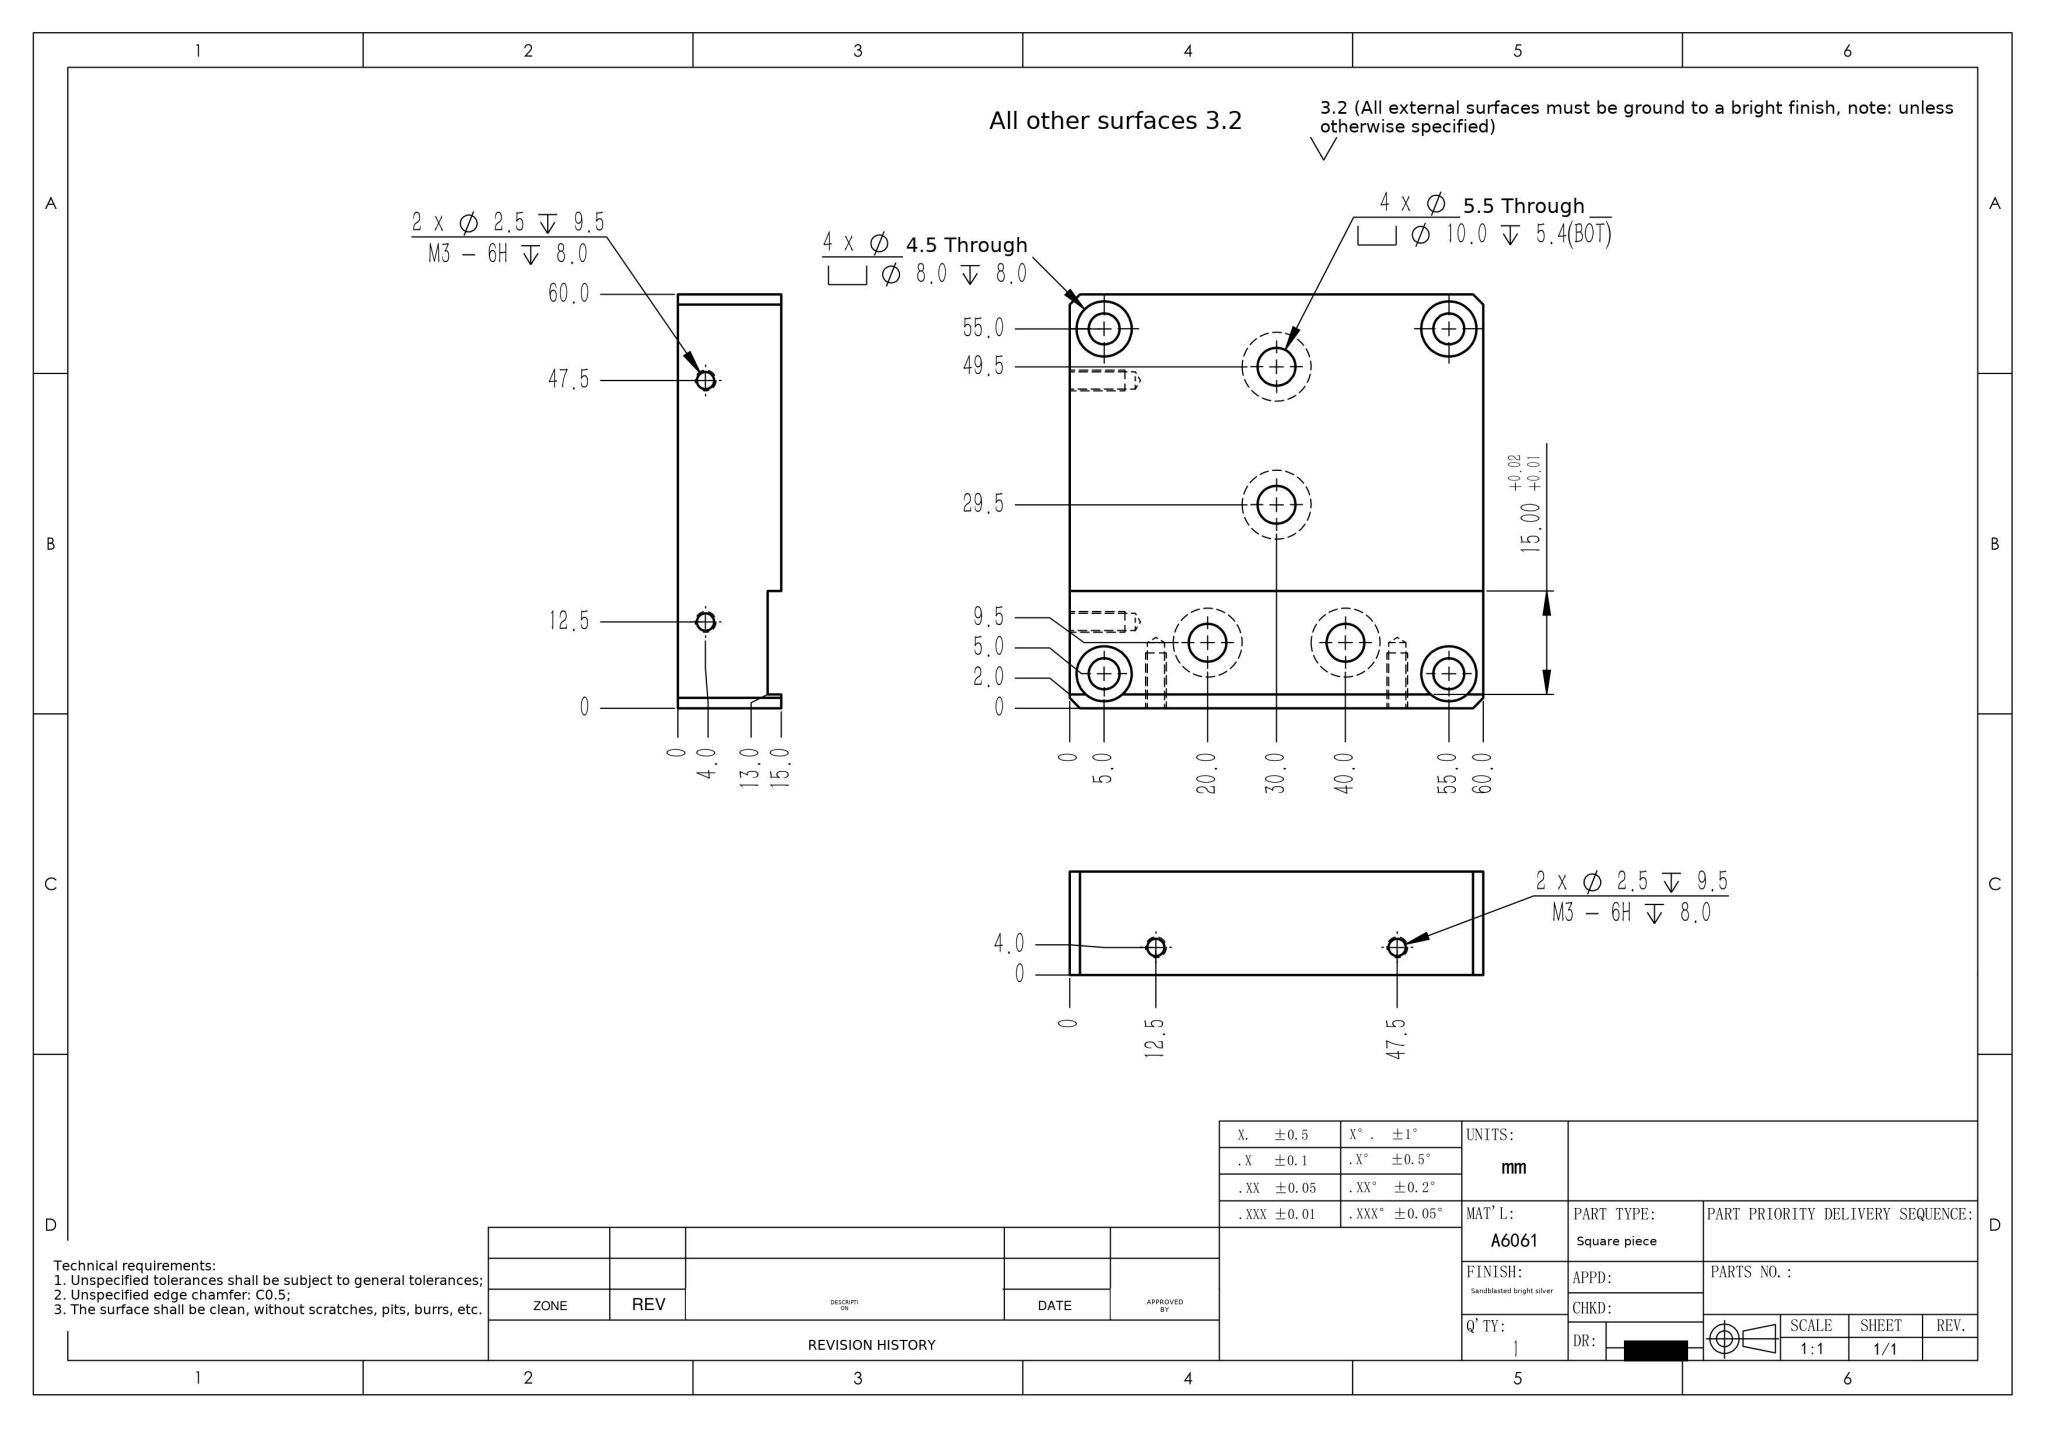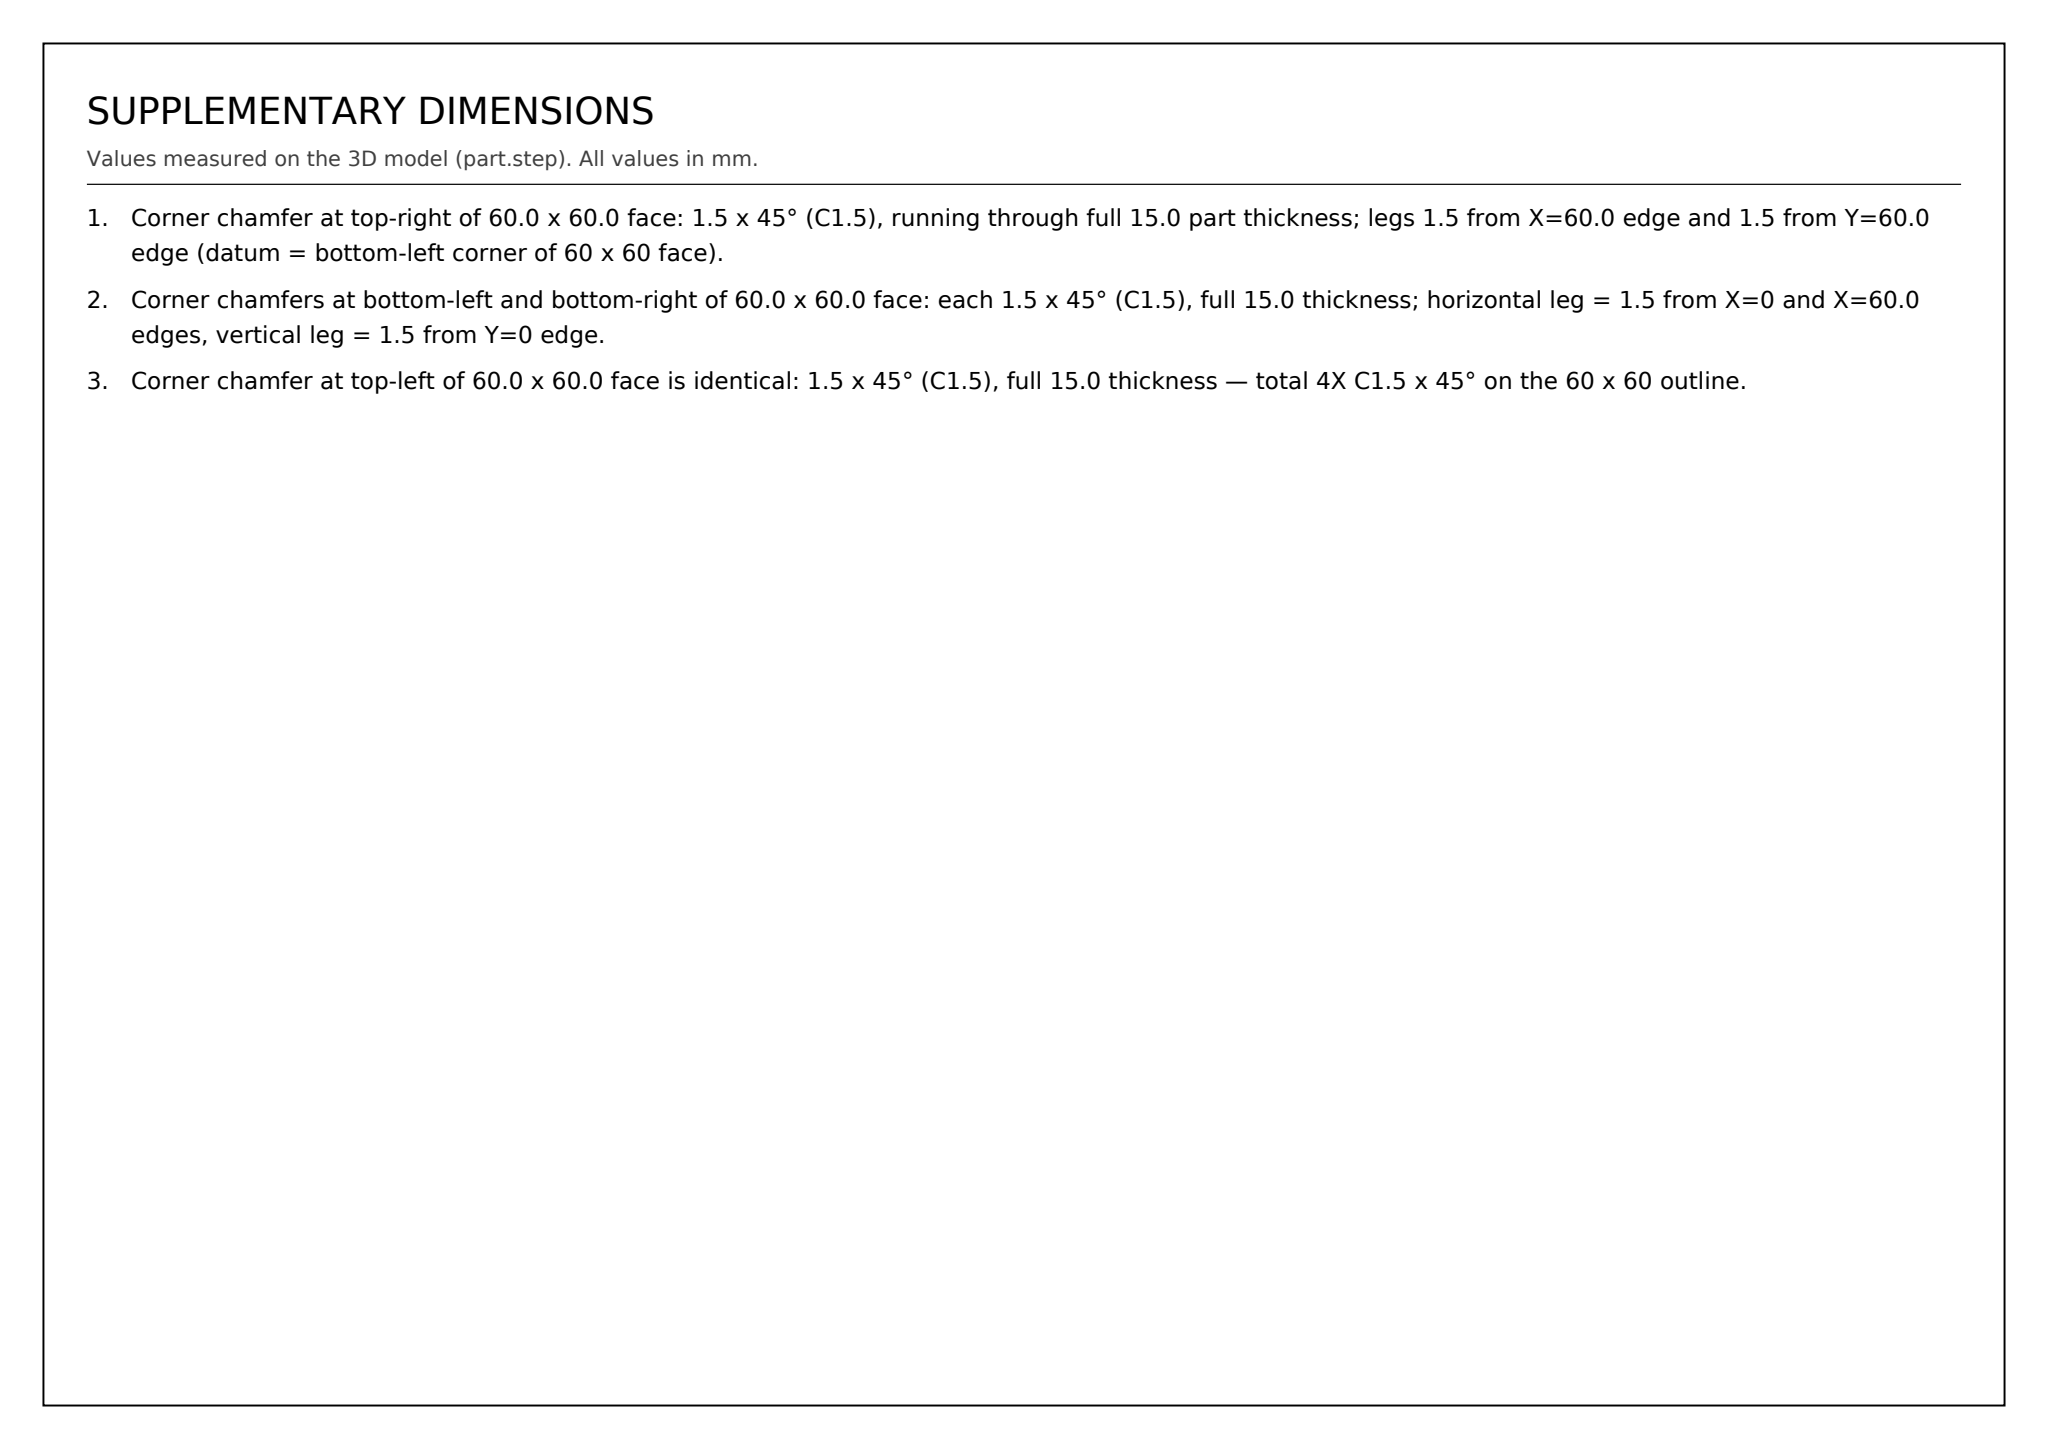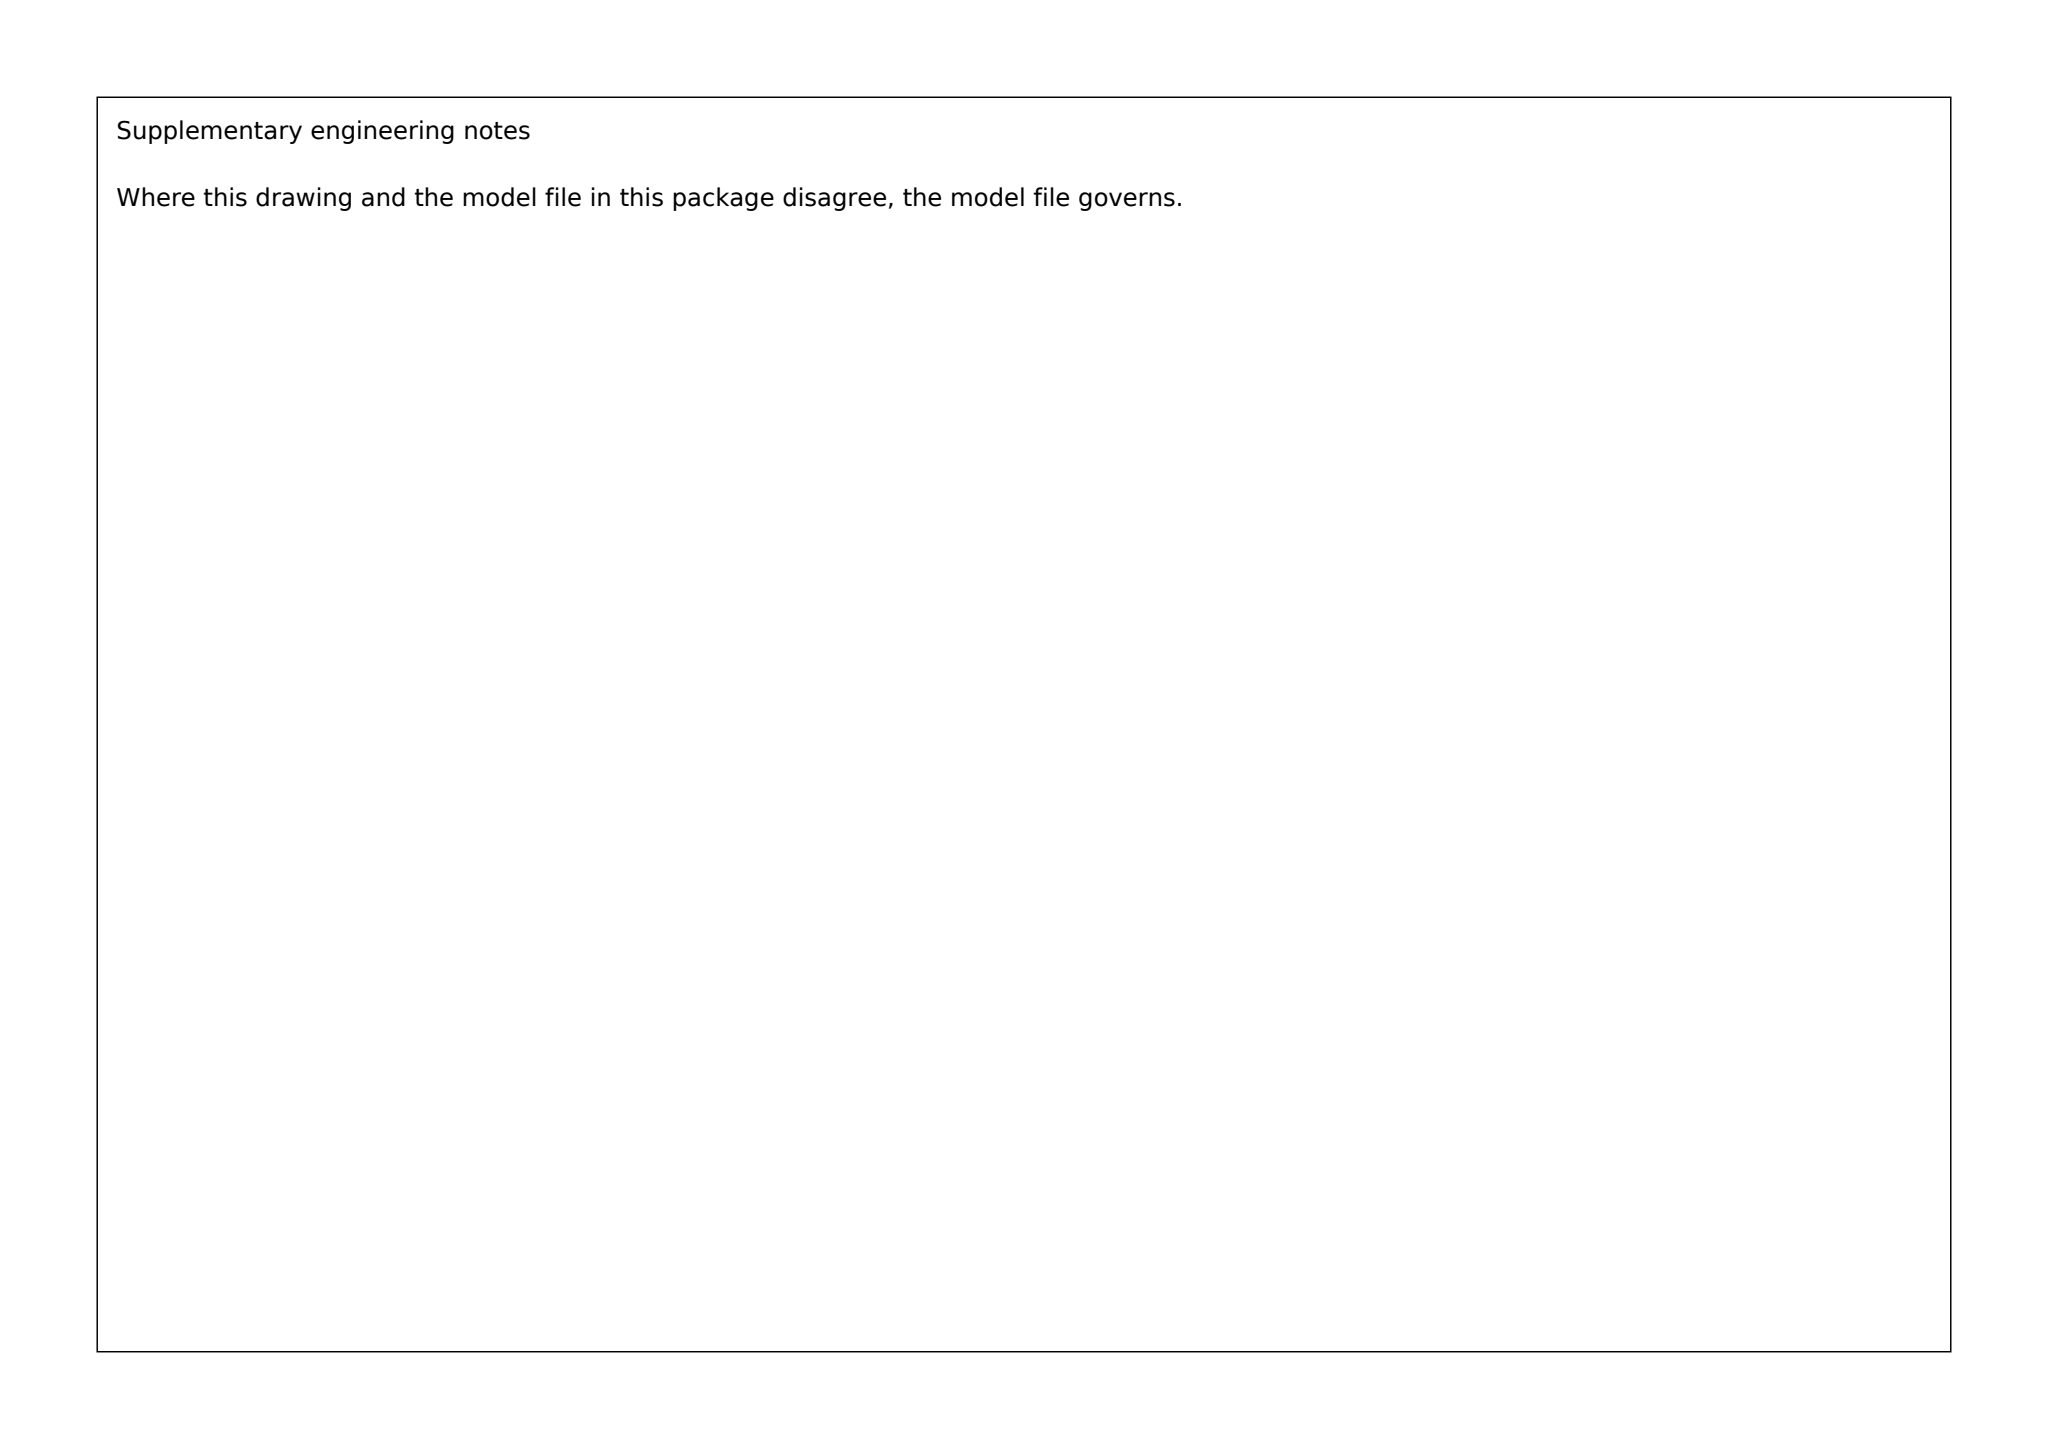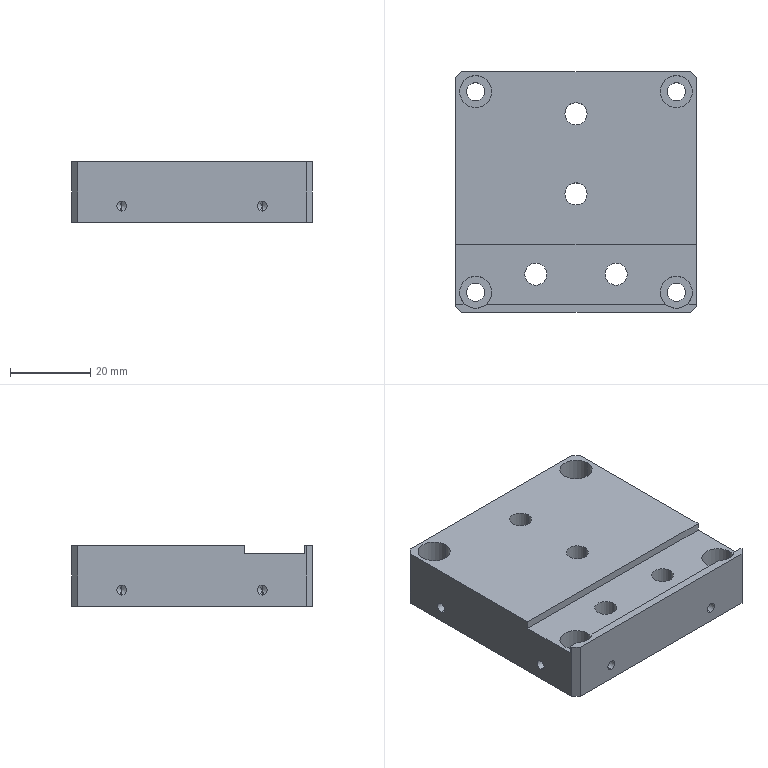Part | SolidWorks | mm | 1 solid | 72 faces | box 60 x 60 x 15 mm | volume 47560 mm3 | cylinder 40 | plane 24 | cone 8 | commonest cylinder face diameters 2.5 x8 10 x8 5.5 x8 8 x8 4.5 x8
Drawing notes:
Corner chamfer at top-right of 60.0 x 60.0 face: 1.5 x 45° (C1.5), running through full 15.0 part thickness; legs 1.5 from X=60.0 edge and 1.5 from Y=60.0 edge (datum = bottom-left corner of 60 x 60 face). | from the solid: inclined_planes: angle_to_xyz_axes [45.0,45.0,90.0], bbox_from [58.5,58.5,0.0], size [1.5,1.5,15.0]
Corner chamfers at bottom-left and bottom-right of 60.0 x 60.0 face: each 1.5 x 45° (C1.5), full 15.0 thickness; horizontal leg = 1.5 from X=0 and X=60.0 edges, vertical leg = 1.5 from Y=0 edge. | from the solid: inclined_planes: angle_to_xyz_axes [45.0,45.0,90.0], bbox_from [0.0,0.0,0.0] and [58.5,0.0,0.0], size [1.5,1.5,15.0]
Corner chamfer at top-left of 60.0 x 60.0 face is identical: 1.5 x 45° (C1.5), full 15.0 thickness — total 4X C1.5 x 45° on the 60 x 60 outline. | from the solid: inclined_planes: angle_to_xyz_axes [45.0,45.0,90.0], bbox_from [0.0,58.5,0.0], size [1.5,1.5,15.0] (4 instances total)
build123d program:
from build123d import *

# Parameters (mm, degrees)
SKETCH1_W                                       = 60
SKETCH1_H                                       = 60
BOSS_EXTRUDE1_DEPTH                             = 15
SKETCH2_W                                       = 60
SKETCH2_H                                       = 15
CUT_EXTRUDE1_DEPTH                              = 2
M4_HEX_SOCKET_HEAD_CAP_SCREW_CBORE1_D           = 4.5
M4_HEX_SOCKET_HEAD_CAP_SCREW_CBORE1_CBORE_D     = 8
M4_HEX_SOCKET_HEAD_CAP_SCREW_CBORE1_CBORE_DEPTH = 8
M5_HEX_SOCKET_HEAD_CAP_SCREW_CBORE1_D           = 5.5
M5_HEX_SOCKET_HEAD_CAP_SCREW_CBORE1_CBORE_D     = 10
M5_HEX_SOCKET_HEAD_CAP_SCREW_CBORE1_CBORE_DEPTH = 5.4
M3_TAPPED_HOLE1_D                               = 2.5
M3_TAPPED_HOLE1_DEPTH                           = 9.5
M3_TAPPED_HOLE1_TIP                             = 0.7511
M3_TAPPED_HOLE2_D                               = 2.5
M3_TAPPED_HOLE2_DEPTH                           = 9.5
M3_TAPPED_HOLE2_TIP                             = 0.7511
CHAMFER1_SIZE                                   = 1.5


with BuildPart() as part:
    # Sketch1 → Boss-Extrude1 (new body)
    with BuildSketch(Plane.XY):
        with Locations((0, -30)):
            Rectangle(SKETCH1_W, SKETCH1_H)
    extrude(amount=BOSS_EXTRUDE1_DEPTH)

    # Sketch2 → Cut-Extrude1 (cut)
    with BuildSketch(Plane.XY.offset(15)):
        with Locations((0, -50.5)):
            Rectangle(SKETCH2_W, SKETCH2_H)
    extrude(amount=-CUT_EXTRUDE1_DEPTH, mode=Mode.SUBTRACT)

    # M4 Hex Socket Head Cap Screw CBORE1 (through all)
    with Locations(Plane.XY.offset(15)):
        with Locations((-25, -5), (25, -5), (25, -55), (-25, -55)):
            CounterBoreHole(M4_HEX_SOCKET_HEAD_CAP_SCREW_CBORE1_D / 2, M4_HEX_SOCKET_HEAD_CAP_SCREW_CBORE1_CBORE_D / 2, M4_HEX_SOCKET_HEAD_CAP_SCREW_CBORE1_CBORE_DEPTH)

    # M5 Hex Socket Head Cap Screw CBORE1 (through all)
    with Locations(Plane(origin=(0, 0, 0), x_dir=(-1, 0, 0), z_dir=(0, 0, -1))):
        with Locations((-10, -50.5), (10, -50.5), (0, -10.5), (0, -30.5)):
            CounterBoreHole(M5_HEX_SOCKET_HEAD_CAP_SCREW_CBORE1_D / 2, M5_HEX_SOCKET_HEAD_CAP_SCREW_CBORE1_CBORE_D / 2, M5_HEX_SOCKET_HEAD_CAP_SCREW_CBORE1_CBORE_DEPTH)

    # M3 Tapped Hole1
    with Locations(Plane.ZY.offset(30)):
        with Locations((4, -12.5), (4, -47.5)):
            Hole(M3_TAPPED_HOLE1_D / 2, depth=M3_TAPPED_HOLE1_DEPTH)
            with Locations((0, 0, -(M3_TAPPED_HOLE1_DEPTH + M3_TAPPED_HOLE1_TIP / 2))):  # 118° drill point
                Cone(0, M3_TAPPED_HOLE1_D / 2, M3_TAPPED_HOLE1_TIP, mode=Mode.SUBTRACT)

    # M3 Tapped Hole2
    with Locations(Plane(origin=(0, -60, 0), x_dir=(-1, 0, 0), z_dir=(0, -1, 0))):
        with Locations((17.5, -4), (-17.5, -4)):
            Hole(M3_TAPPED_HOLE2_D / 2, depth=M3_TAPPED_HOLE2_DEPTH)
            with Locations((0, 0, -(M3_TAPPED_HOLE2_DEPTH + M3_TAPPED_HOLE2_TIP / 2))):  # 118° drill point
                Cone(0, M3_TAPPED_HOLE2_D / 2, M3_TAPPED_HOLE2_TIP, mode=Mode.SUBTRACT)

    # Chamfer1
    chamfer1_edges = [part.edges().sort_by_distance(p)[0] for p in [
        (-30, 0, 7.5),
        (30, 0, 7.5),
        (30, -60, 7.5),
        (-30, -60, 7.5),
    ]]
    chamfer(chamfer1_edges, length=CHAMFER1_SIZE)


solid = part.part